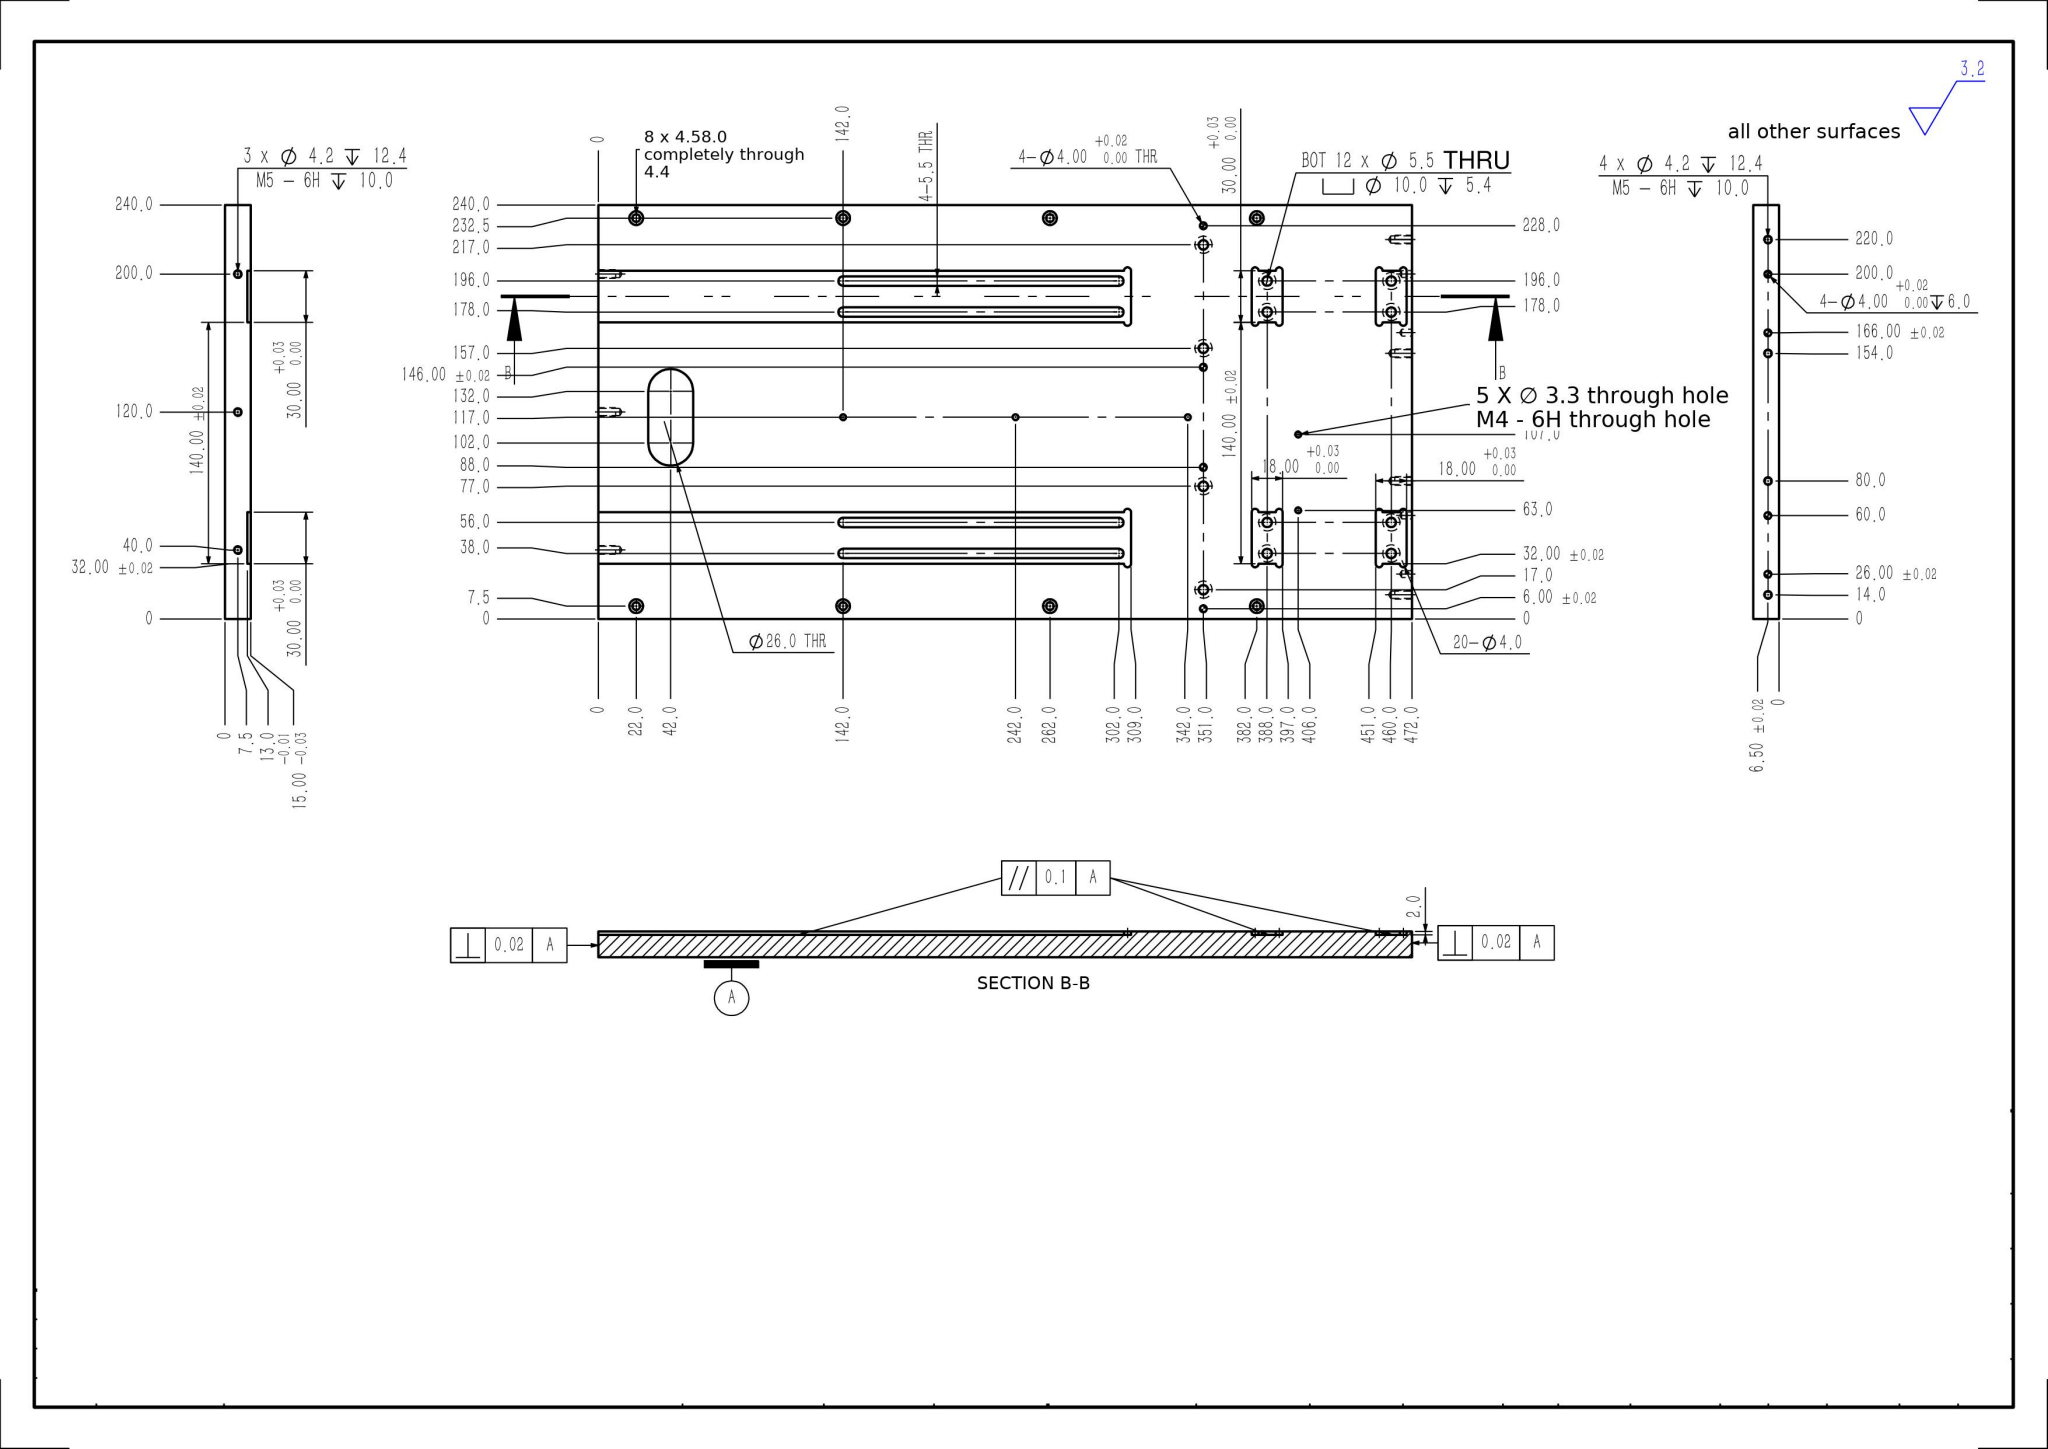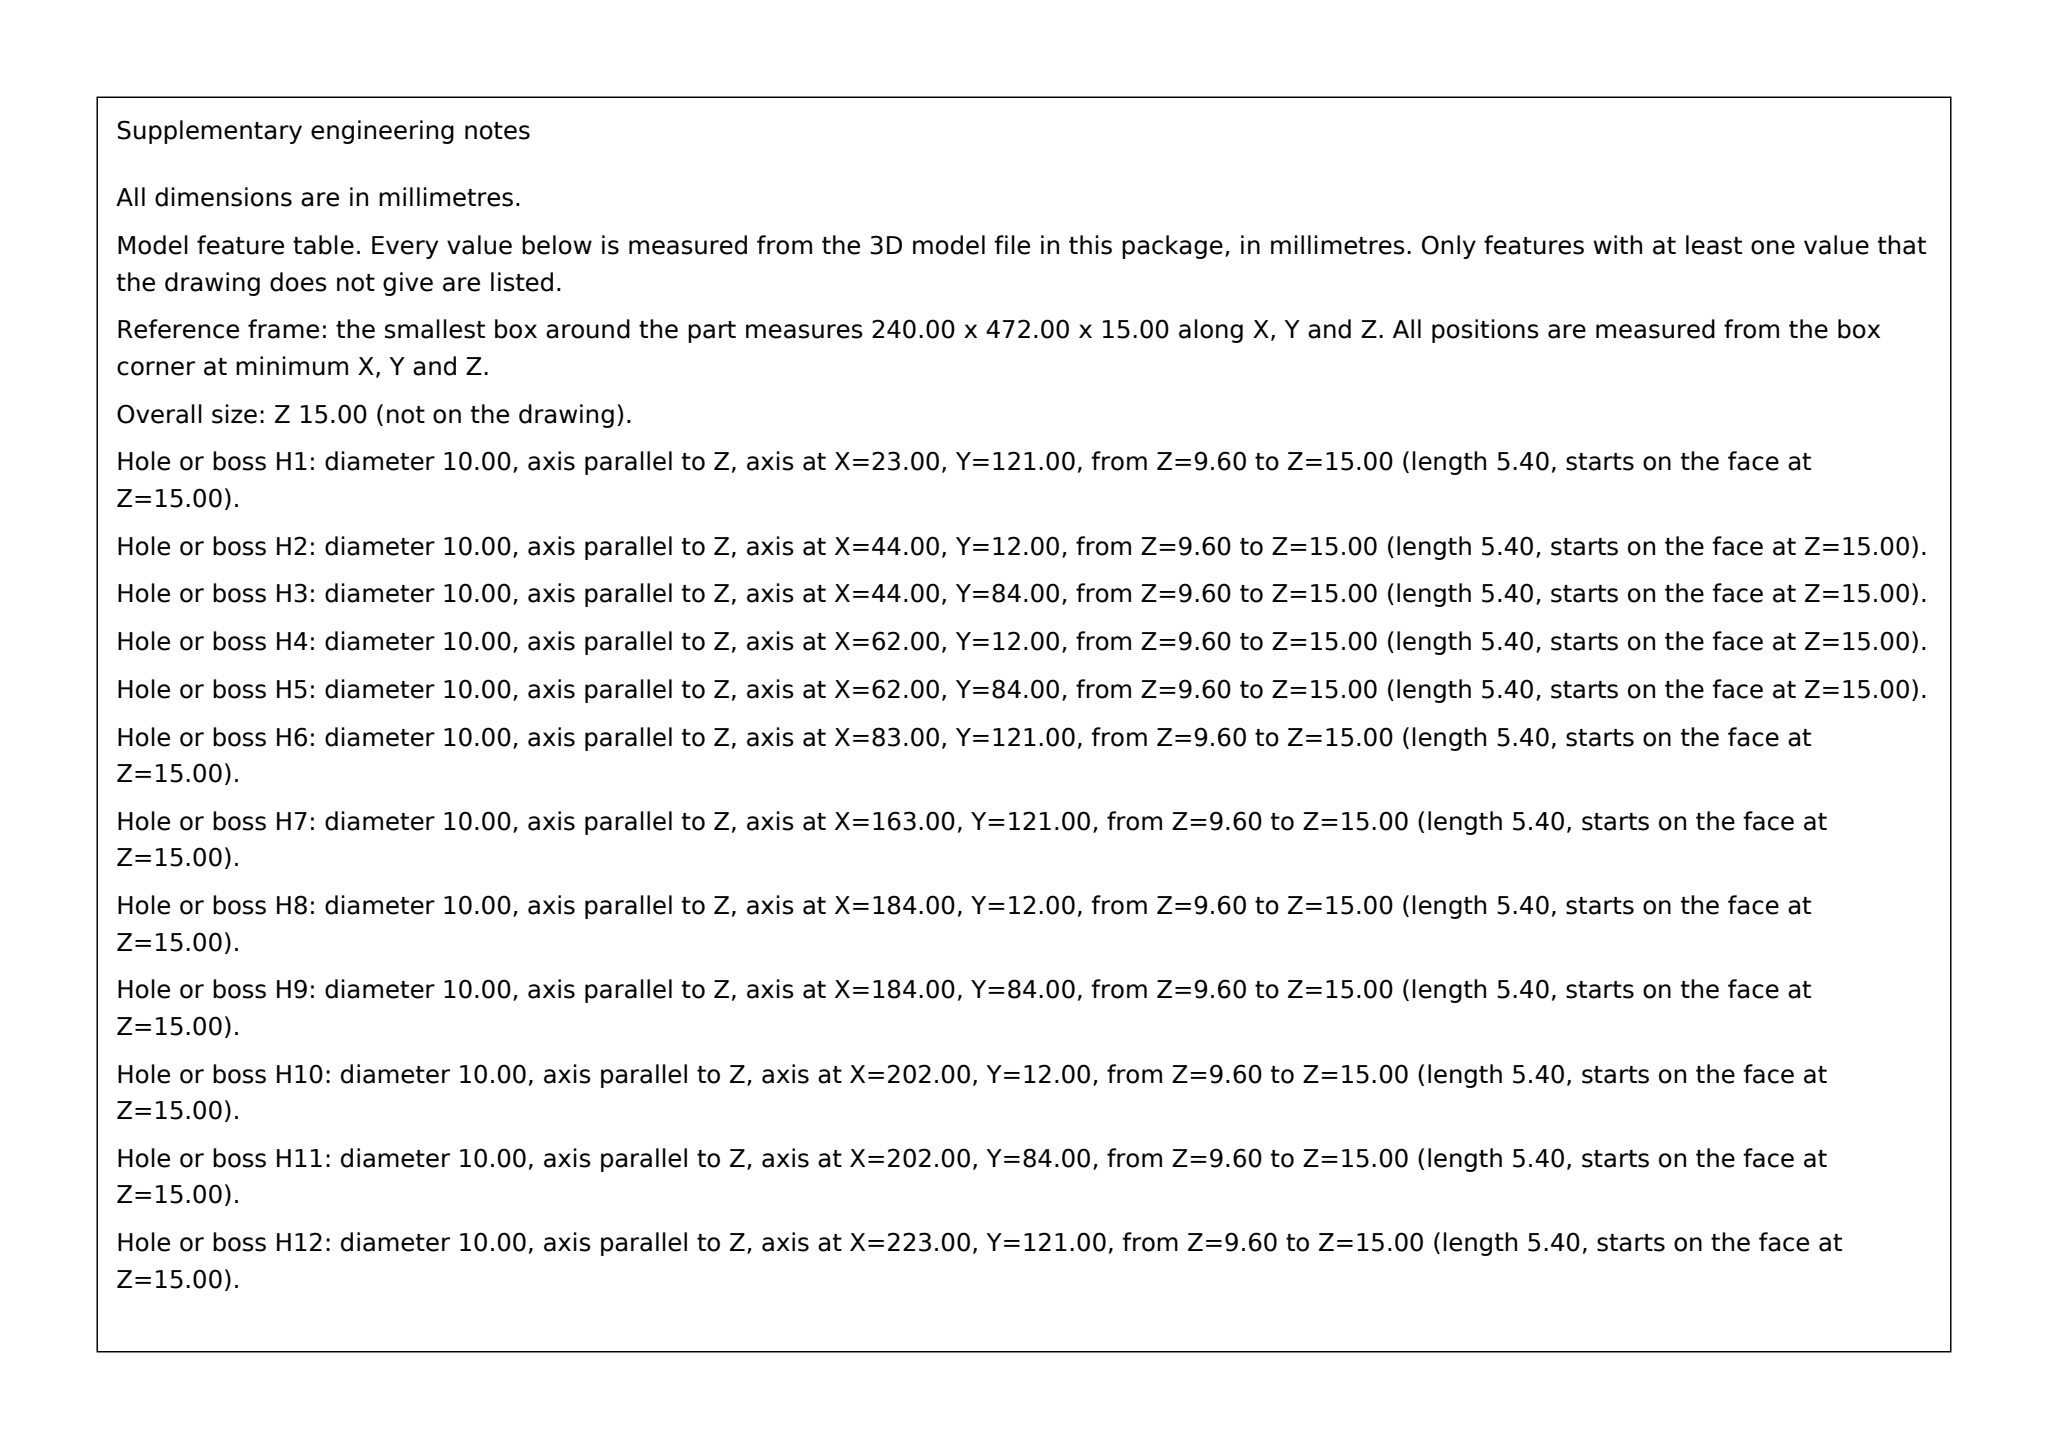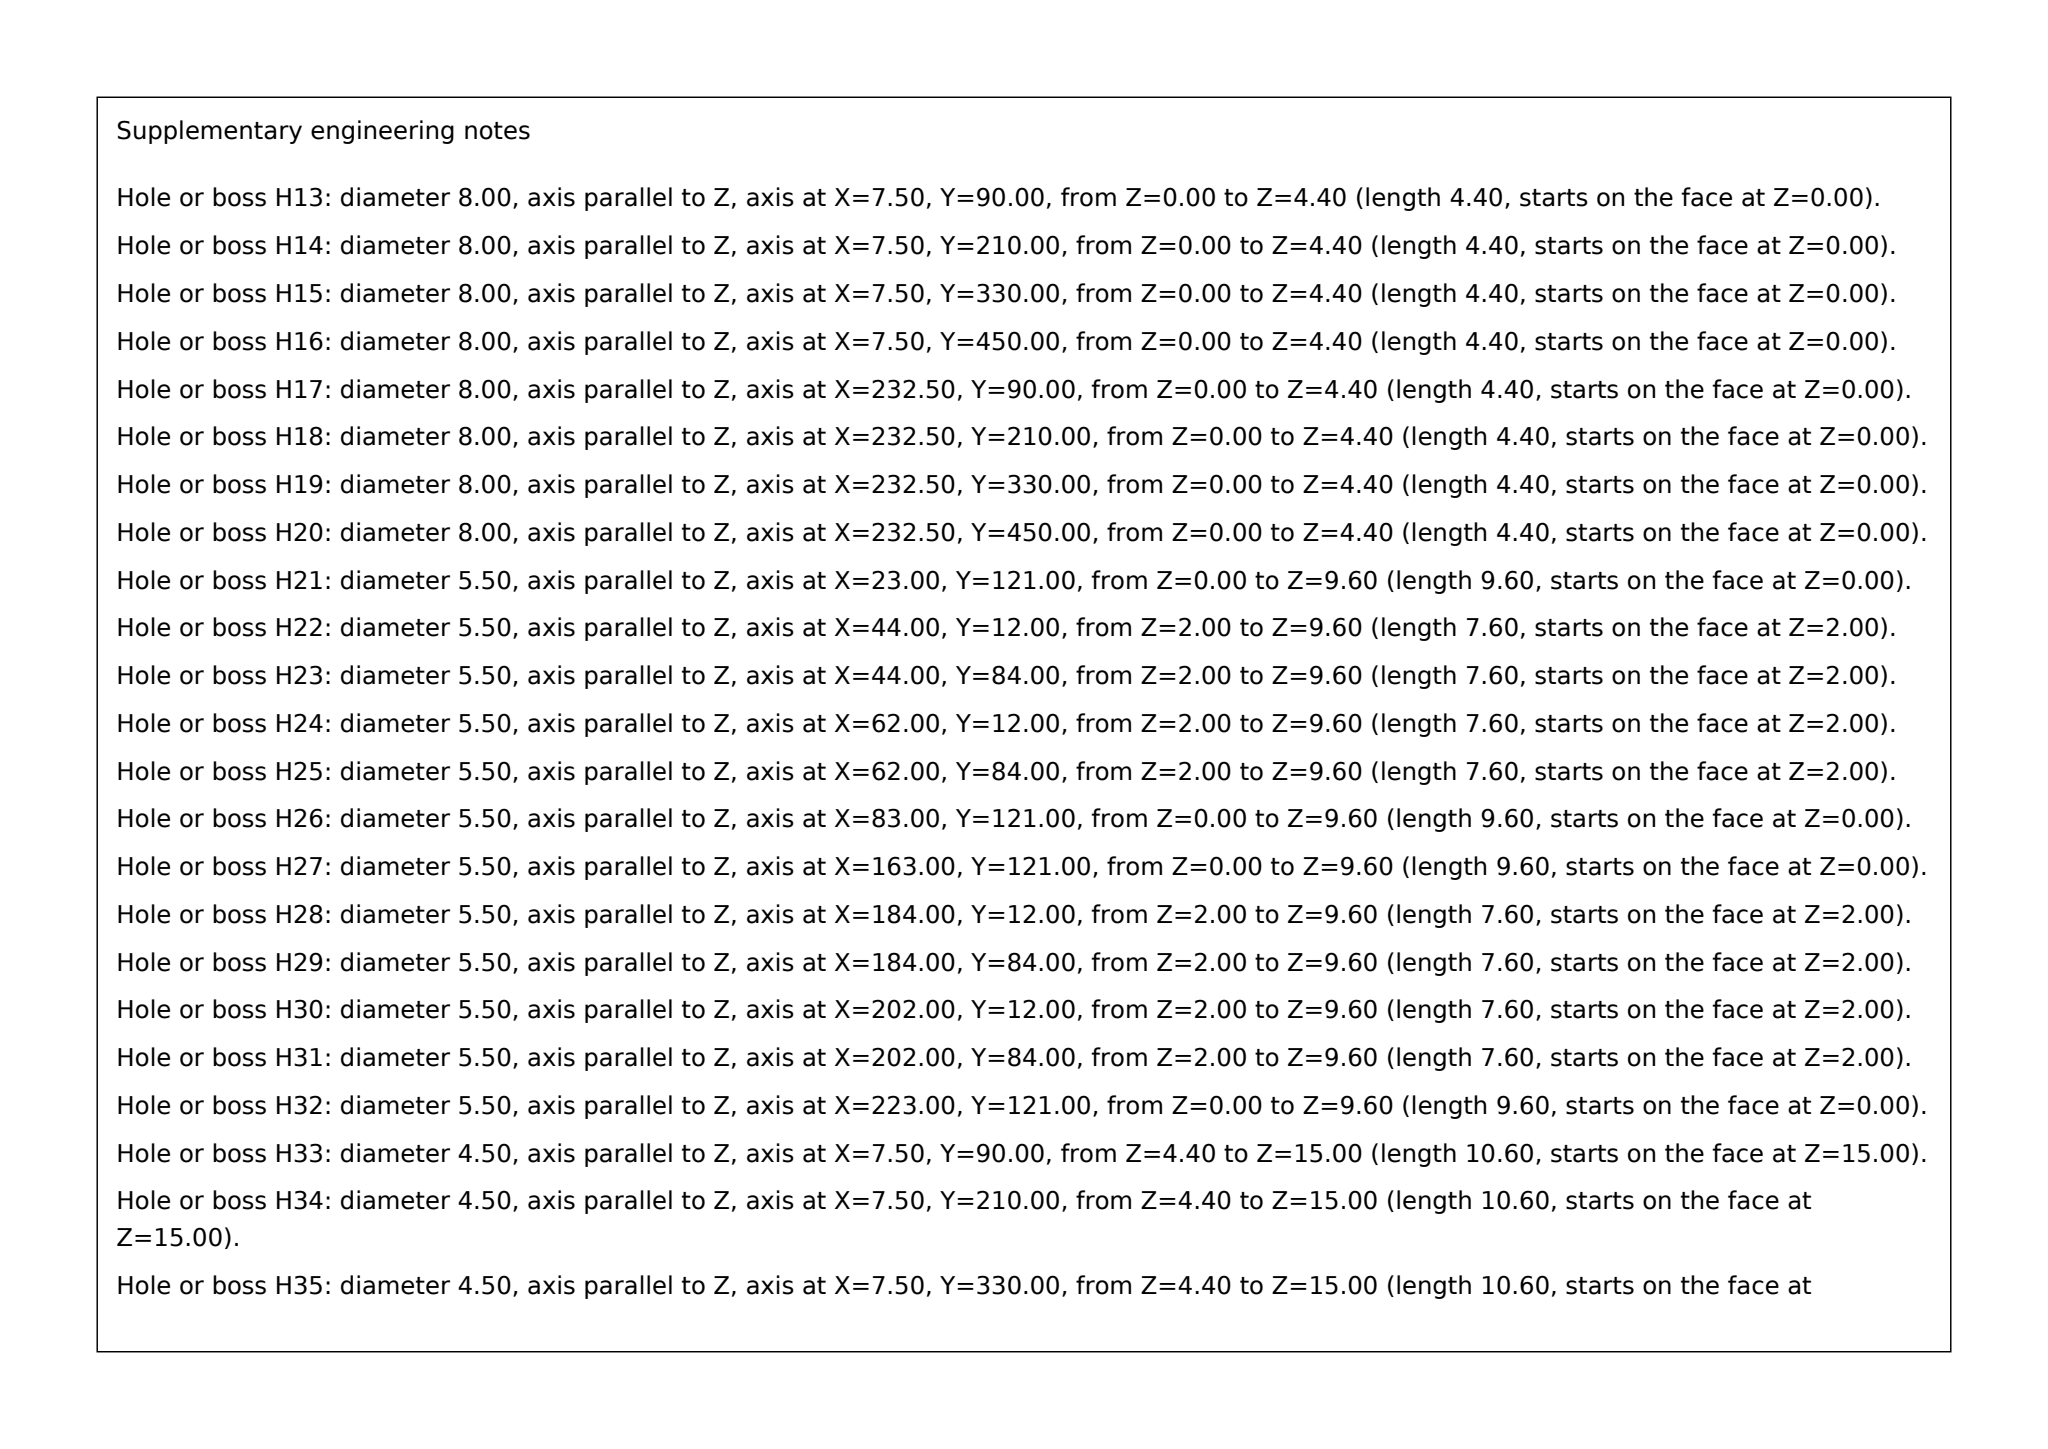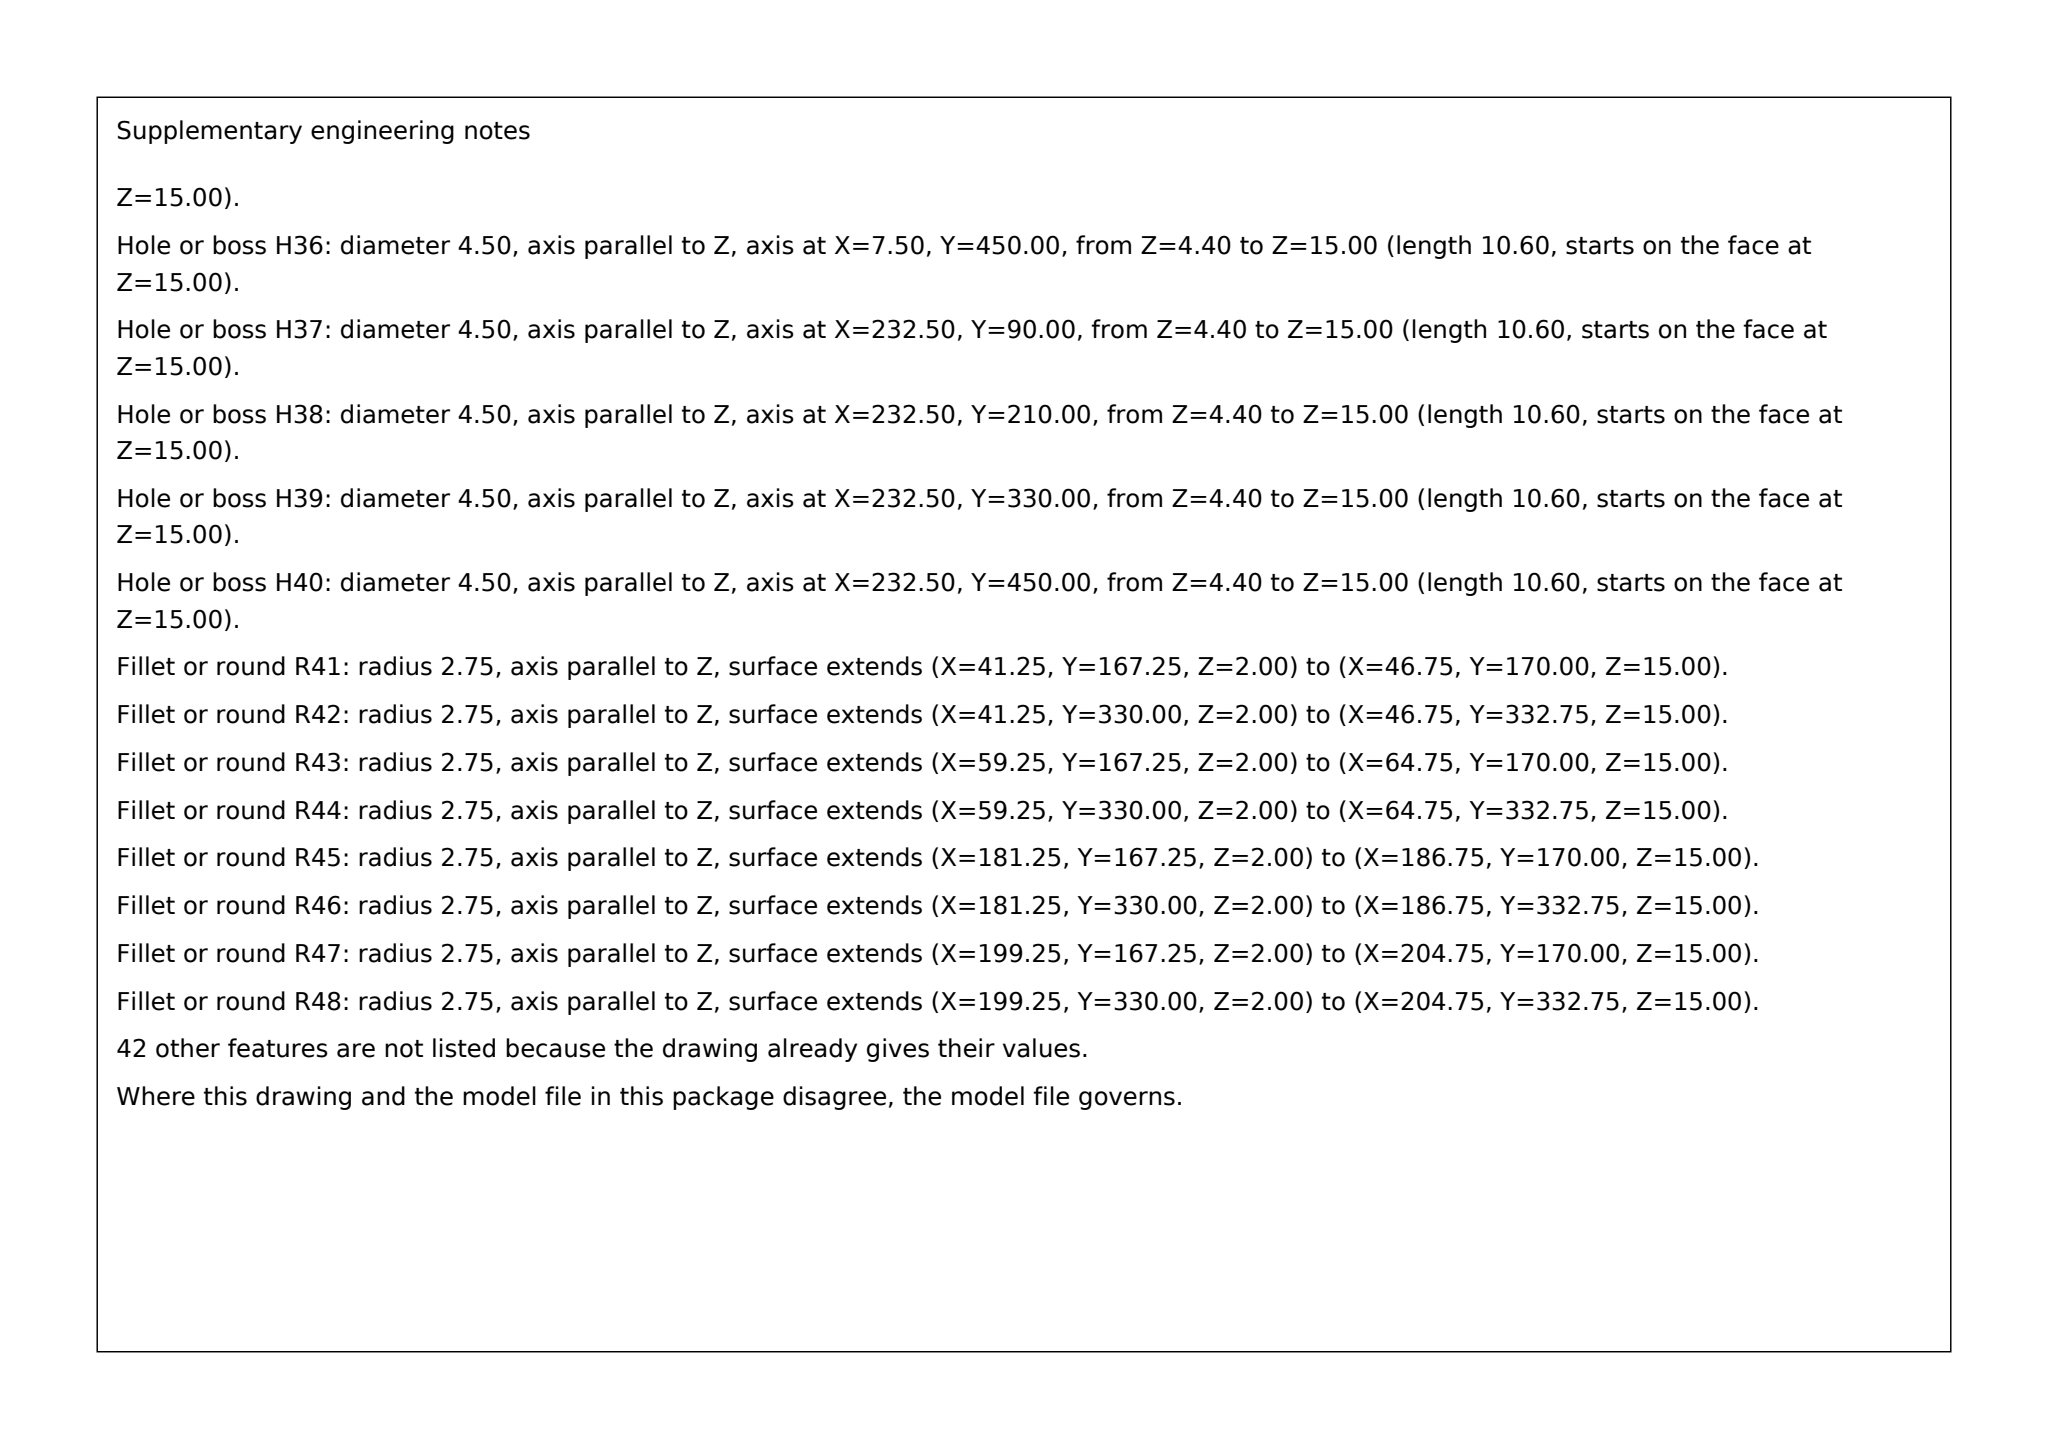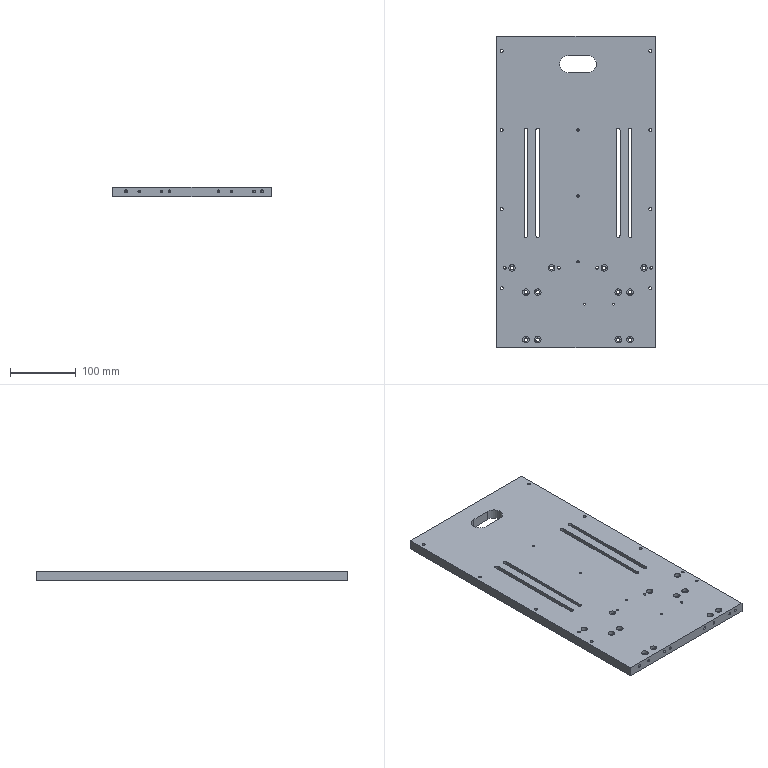Part | SolidWorks | mm | 1 solid | 247 faces | box 240 x 472 x 15 mm | volume 1577365 mm3 | cylinder 161 | plane 64 | cone 22 | commonest cylinder face diameters 4 x46 5.5 x32 10 x24 8 x16 4.5 x16 4.2 x14 3.3 x10 26 x3
build123d program:
from build123d import *

# Parameters (mm, degrees)
SKETCH1_W                                       = 240
SKETCH1_H                                       = 472
BOSS_EXTRUDE1_DEPTH                             = 7.5
SKETCH2_W                                       = 30
SKETCH2_H                                       = 18
SKETCH2_H_2                                     = 309
CUT_EXTRUDE1_DEPTH                              = 2
SKETCH3_R                                       = 2
CUT_EXTRUDE2_DEPTH                              = 2
LPATTERN1_COUNT                                 = 2
LPATTERN1_PITCH                                 = 140
M5_TAPPED_HOLE1_D                               = 4.2
M5_TAPPED_HOLE1_DEPTH                           = 12.4
M5_TAPPED_HOLE1_TIP                             = 1.262
M4_HEX_SOCKET_HEAD_CAP_SCREW_CBORE1_D           = 4.5
M4_HEX_SOCKET_HEAD_CAP_SCREW_CBORE1_CBORE_D     = 8
M4_HEX_SOCKET_HEAD_CAP_SCREW_CBORE1_CBORE_DEPTH = 4.4
M4_TAPPED_HOLE1_D                               = 3.3
M5_TAPPED_HOLE2_D                               = 4.2
M5_TAPPED_HOLE2_DEPTH                           = 12.4
M5_TAPPED_HOLE2_TIP                             = 1.262
SIZE_MM_DOWEL_PIN_HOLE1_D                       = 4
SIZE_MM_DOWEL_PIN_HOLE1_DEPTH                   = 6
SIZE_MM_DOWEL_PIN_HOLE1_TIP                     = 1.202
M5_HEX_SOCKET_HEAD_CAP_SCREW_CBORE1_D           = 5.5
M5_HEX_SOCKET_HEAD_CAP_SCREW_CBORE1_CBORE_D     = 10
M5_HEX_SOCKET_HEAD_CAP_SCREW_CBORE1_CBORE_DEPTH = 5.4
CUT_EXTRUDE3_DEPTH                              = 266.181
M4_TAPPED_HOLE2_D                               = 3.3
M5_HEX_SOCKET_HEAD_CAP_SCREW_CBORE2_D           = 5.5
M5_HEX_SOCKET_HEAD_CAP_SCREW_CBORE2_CBORE_D     = 10
M5_HEX_SOCKET_HEAD_CAP_SCREW_CBORE2_CBORE_DEPTH = 5.4
CUT_EXTRUDE4_DEPTH                              = 266.181
SIZE_MM_DOWEL_PIN_HOLE2_D                       = 4


with BuildPart() as part:
    # Sketch1 → Boss-Extrude1 (new, symmetric)
    with BuildSketch(Plane.XY):
        Rectangle(SKETCH1_W, SKETCH1_H)
    extrude(amount=BOSS_EXTRUDE1_DEPTH, both=True)

    # Sketch2 → Cut-Extrude1 (cut)
    with BuildSketch(Plane(origin=(0, 0, -7.5), x_dir=(-1, 0, 0), z_dir=(0, 0, -1))):
        with Locations((-73, -224)):
            Rectangle(SKETCH2_W, SKETCH2_H)
        with Locations((-73, -152)):
            Rectangle(SKETCH2_W, SKETCH2_H)
        with Locations((-73, 81.5)):
            Rectangle(SKETCH2_W, SKETCH2_H_2)
    cut_extrude1 = extrude(amount=-CUT_EXTRUDE1_DEPTH, mode=Mode.SUBTRACT)

    # Sketch3 → Cut-Extrude2 (cut)
    with BuildSketch(Plane(origin=(0, 0, -7.5), x_dir=(-1, 0, 0), z_dir=(0, 0, -1))):
        with Locations((-58, -231)):
            Circle(SKETCH3_R)
        with Locations((-88, -231)):
            Circle(SKETCH3_R)
        with Locations((-58, -217)):
            Circle(SKETCH3_R)
        with Locations((-88, -217)):
            Circle(SKETCH3_R)
        with Locations((-58, -159)):
            Circle(SKETCH3_R)
        with Locations((-88, -159)):
            Circle(SKETCH3_R)
        with Locations((-58, -145)):
            Circle(SKETCH3_R)
        with Locations((-88, -145)):
            Circle(SKETCH3_R)
        with Locations((-58, -71)):
            Circle(SKETCH3_R)
        with Locations((-88, -71)):
            Circle(SKETCH3_R)
    cut_extrude2 = extrude(amount=-CUT_EXTRUDE2_DEPTH, mode=Mode.SUBTRACT)

    # LPattern1: Cut-Extrude1, Cut-Extrude2 ×2
    with Locations(*[(-i * LPATTERN1_PITCH, 0, 0) for i in range(1, LPATTERN1_COUNT)]):
        add(cut_extrude1, mode=Mode.SUBTRACT)
        add(cut_extrude2, mode=Mode.SUBTRACT)

    # M5 Tapped Hole1
    with Locations(Plane(origin=(0, 236, 0), x_dir=(1, 0, 0), z_dir=(0, 1, 0))):
        with Locations((-80, 0), (80, 0), (0, 0)):
            Hole(M5_TAPPED_HOLE1_D / 2, depth=M5_TAPPED_HOLE1_DEPTH)
            with Locations((0, 0, -(M5_TAPPED_HOLE1_DEPTH + M5_TAPPED_HOLE1_TIP / 2))):  # 118° drill point
                Cone(0, M5_TAPPED_HOLE1_D / 2, M5_TAPPED_HOLE1_TIP, mode=Mode.SUBTRACT)

    # M4 Hex Socket Head Cap Screw CBORE1 (through all)
    with Locations(Plane(origin=(0, 0, -7.5), x_dir=(-1, 0, 0), z_dir=(0, 0, -1))):
        with Locations((112.5, -146), (112.5, -26), (112.5, 94), (112.5, 214), (-112.5, 214), (-112.5, 94), (-112.5, -26), (-112.5, -146)):
            CounterBoreHole(M4_HEX_SOCKET_HEAD_CAP_SCREW_CBORE1_D / 2, M4_HEX_SOCKET_HEAD_CAP_SCREW_CBORE1_CBORE_D / 2, M4_HEX_SOCKET_HEAD_CAP_SCREW_CBORE1_CBORE_DEPTH)

    # M4 Tapped Hole1 (through all)
    with Locations(Plane.XY.offset(7.5)):
        with Locations((57, -170), (13, -170)):
            Hole(M4_TAPPED_HOLE1_D / 2)

    # M5 Tapped Hole2
    with Locations(Plane(origin=(0, -236, 0), x_dir=(-1, 0, 0), z_dir=(0, -1, 0))):
        with Locations((-106, -1), (-40, -1), (34, -1), (100, -1)):
            Hole(M5_TAPPED_HOLE2_D / 2, depth=M5_TAPPED_HOLE2_DEPTH)
            with Locations((0, 0, -(M5_TAPPED_HOLE2_DEPTH + M5_TAPPED_HOLE2_TIP / 2))):  # 118° drill point
                Cone(0, M5_TAPPED_HOLE2_D / 2, M5_TAPPED_HOLE2_TIP, mode=Mode.SUBTRACT)

    # Size mm Dowel Pin Hole1
    with Locations(Plane(origin=(0, -236, 0), x_dir=(-1, 0, 0), z_dir=(0, -1, 0))):
        with Locations((-94, -1), (-60, -1), (46, -1), (80, -1)):
            Hole(SIZE_MM_DOWEL_PIN_HOLE1_D / 2, depth=SIZE_MM_DOWEL_PIN_HOLE1_DEPTH)
            with Locations((0, 0, -(SIZE_MM_DOWEL_PIN_HOLE1_DEPTH + SIZE_MM_DOWEL_PIN_HOLE1_TIP / 2))):  # 118° drill point
                Cone(0, SIZE_MM_DOWEL_PIN_HOLE1_D / 2, SIZE_MM_DOWEL_PIN_HOLE1_TIP, mode=Mode.SUBTRACT)

    # M5 Hex Socket Head Cap Screw CBORE1 (through all)
    with Locations(Plane.XY.offset(7.5)):
        with Locations((82, -224), (64, -224), (82, -152), (64, -152), (-58, -224), (-76, -224), (-58, -152), (-76, -152)):
            CounterBoreHole(M5_HEX_SOCKET_HEAD_CAP_SCREW_CBORE1_D / 2, M5_HEX_SOCKET_HEAD_CAP_SCREW_CBORE1_CBORE_D / 2, M5_HEX_SOCKET_HEAD_CAP_SCREW_CBORE1_CBORE_DEPTH)

    # Sketch21 → Cut-Extrude3 (cut, through all)
    with BuildSketch(Plane.XY.offset(7.5)):
        with BuildLine():
            Line((79.25, -66), (79.25, 94))
            ThreePointArc((79.25, 94), (82, 96.75), (84.75, 94))
            Line((84.75, 94), (84.75, -66))
            ThreePointArc((84.75, -66), (82, -68.75), (79.25, -66))
        make_face()
        with BuildLine():
            Line((66.75, -66), (66.75, 94))
            ThreePointArc((66.75, 94), (64, 96.75), (61.25, 94))
            Line((61.25, 94), (61.25, -66))
            ThreePointArc((61.25, -66), (64, -68.75), (66.75, -66))
        make_face()
        with BuildLine():
            Line((-60.75, -66), (-60.75, 94))
            ThreePointArc((-60.75, 94), (-58, 96.75), (-55.25, 94))
            Line((-55.25, 94), (-55.25, -66))
            ThreePointArc((-55.25, -66), (-58, -68.75), (-60.75, -66))
        make_face()
        with BuildLine():
            Line((-73.25, -66), (-73.25, 94))
            ThreePointArc((-73.25, 94), (-76, 96.75), (-78.75, 94))
            Line((-78.75, 94), (-78.75, -66))
            ThreePointArc((-78.75, -66), (-76, -68.75), (-73.25, -66))
        make_face()
    extrude(amount=-CUT_EXTRUDE3_DEPTH, mode=Mode.SUBTRACT)

    # M4 Tapped Hole2 (through all)
    with Locations(Plane.XY.offset(7.5)):
        with Locations((3, -106), (3, -6), (3, 94), (3, 194)):
            Hole(M4_TAPPED_HOLE2_D / 2)

    # M5 Hex Socket Head Cap Screw CBORE2 (through all)
    with Locations(Plane.XY.offset(7.5)):
        with Locations((103, -115), (43, -115), (-37, -115), (-97, -115)):
            CounterBoreHole(M5_HEX_SOCKET_HEAD_CAP_SCREW_CBORE2_D / 2, M5_HEX_SOCKET_HEAD_CAP_SCREW_CBORE2_CBORE_D / 2, M5_HEX_SOCKET_HEAD_CAP_SCREW_CBORE2_CBORE_DEPTH)

    # Sketch26 → Cut-Extrude4 (cut, through all)
    with BuildSketch(Plane(origin=(0, 0, -7.5), x_dir=(-1, 0, 0), z_dir=(0, 0, -1))):
        with BuildLine():
            Line((-18, 207), (12, 207))
            ThreePointArc((12, 207), (25, 194), (12, 181))
            Line((12, 181), (-18, 181))
            ThreePointArc((-18, 181), (-31, 194), (-18, 207))
        make_face()
    extrude(amount=-CUT_EXTRUDE4_DEPTH, mode=Mode.SUBTRACT)

    # Size mm Dowel Pin Hole2 (through all)
    with Locations(Plane.XY.offset(7.5)):
        with Locations((114, -115), (32, -115), (-26, -115), (-108, -115)):
            Hole(SIZE_MM_DOWEL_PIN_HOLE2_D / 2)


solid = part.part